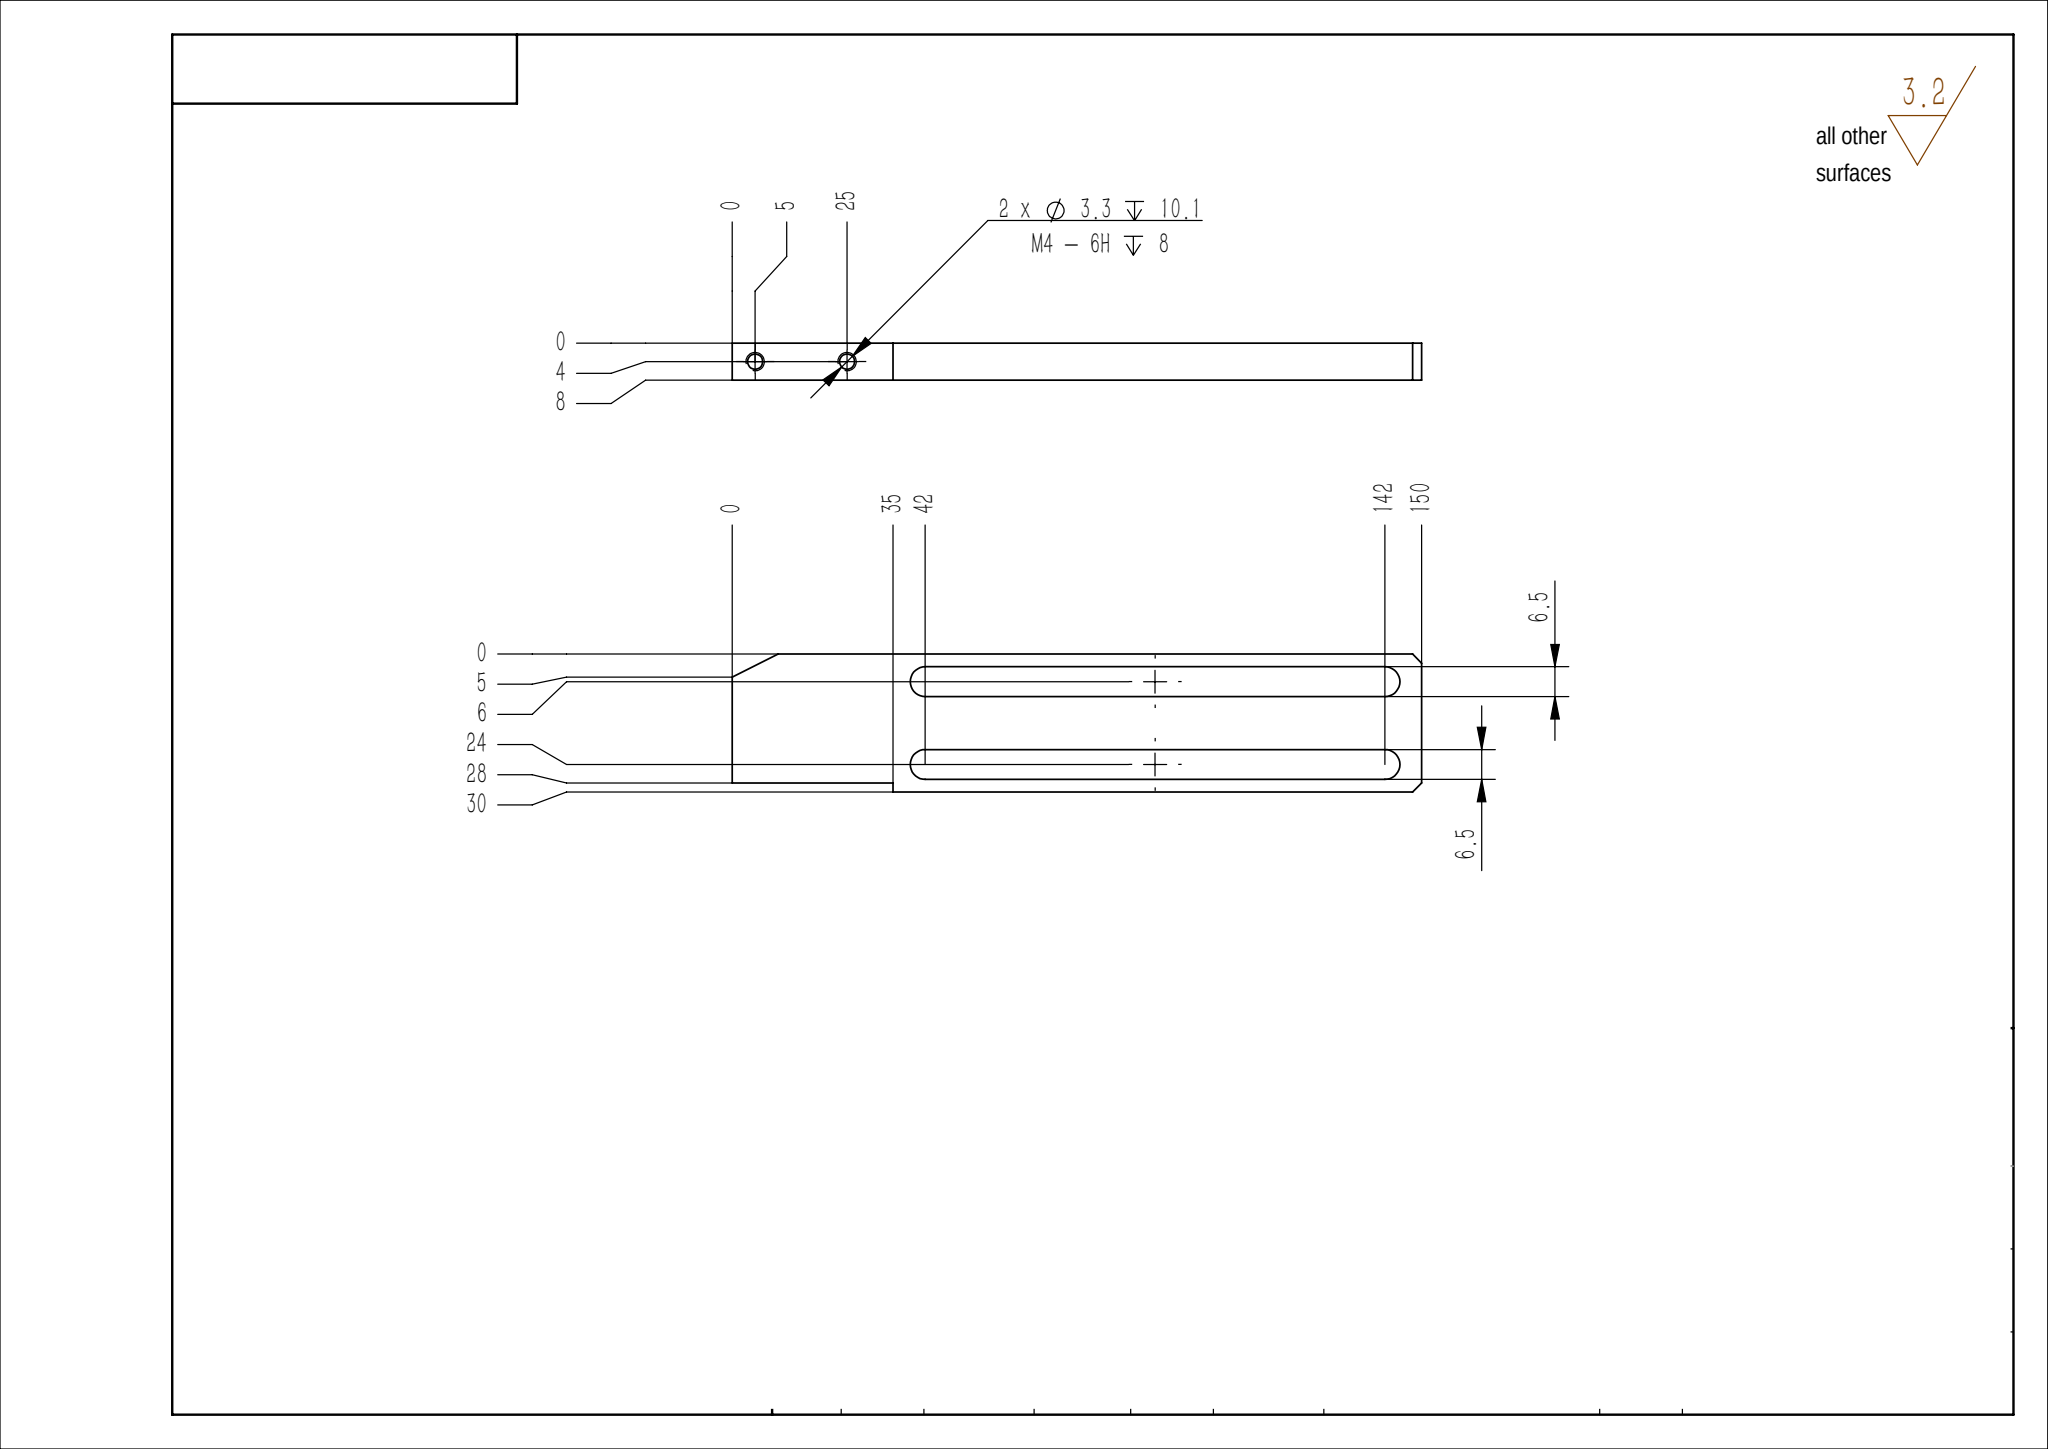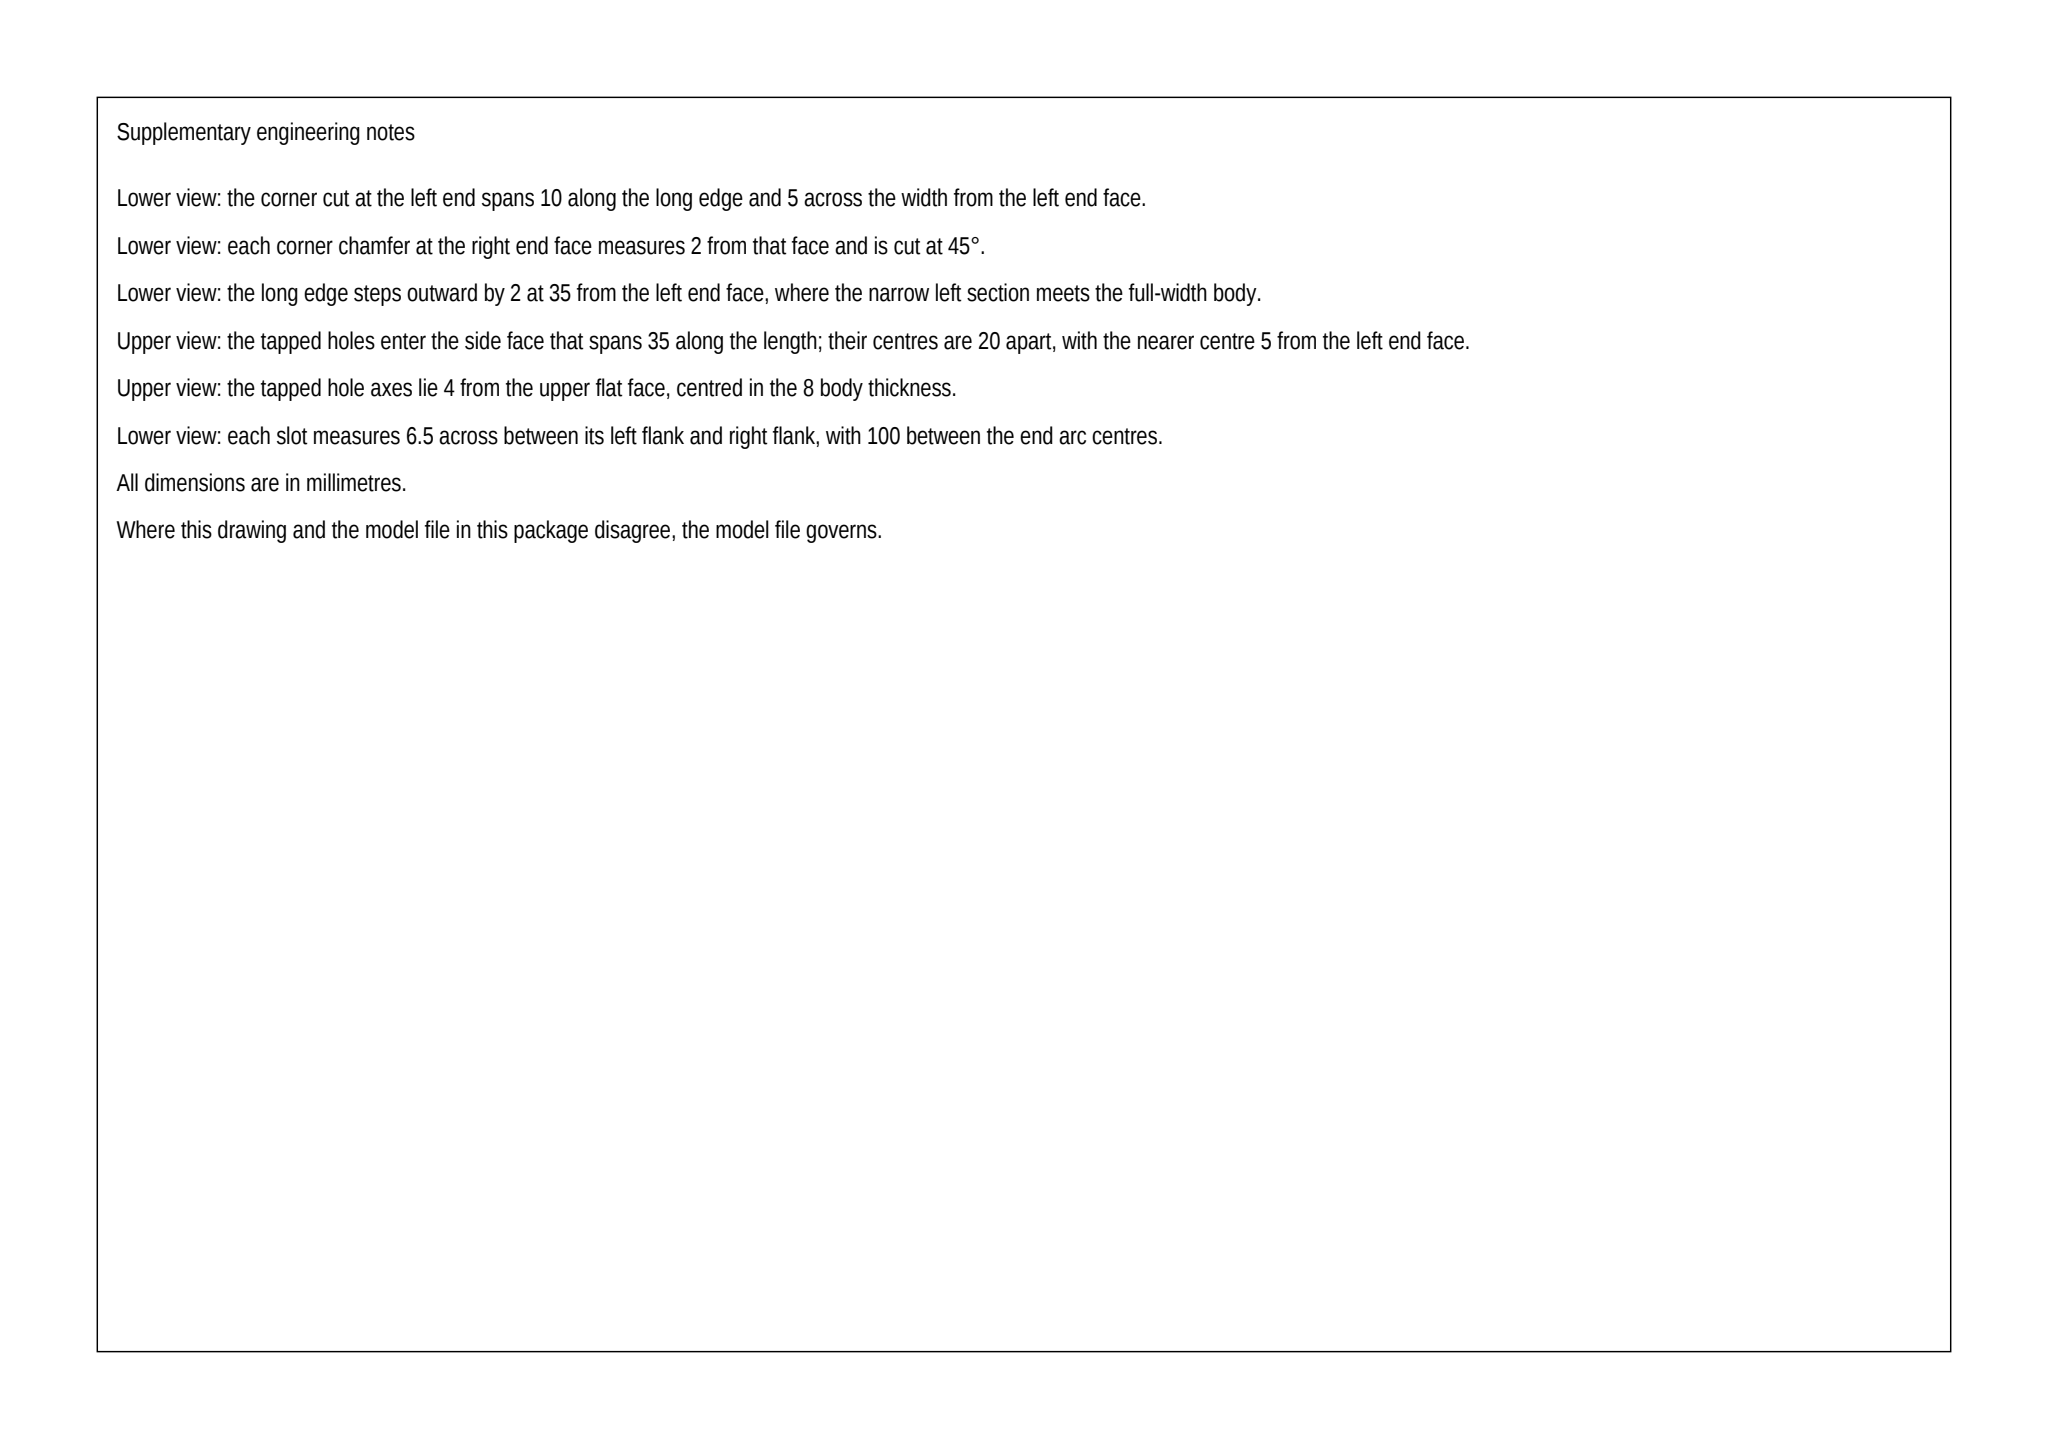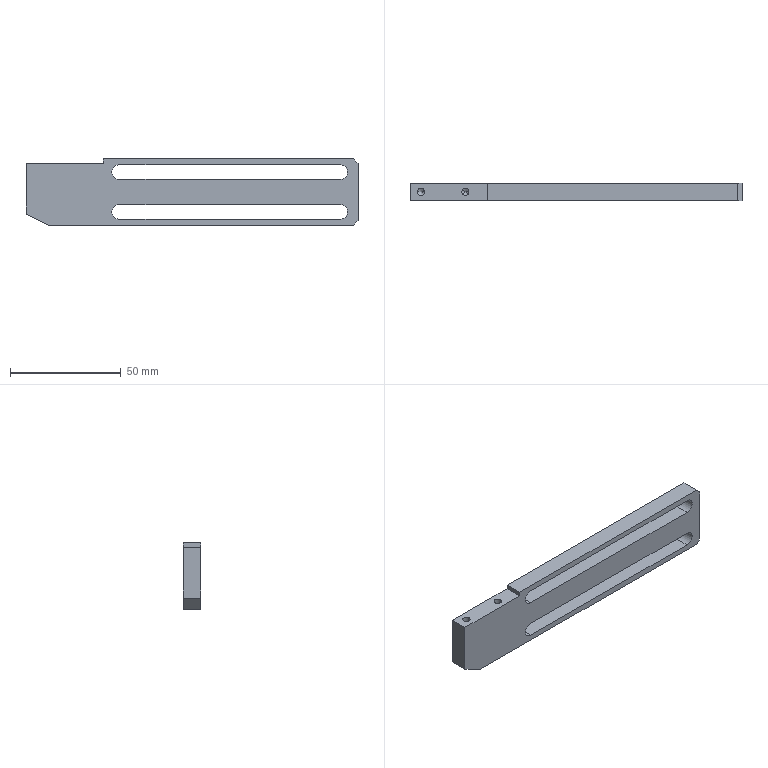Part | SolidWorks | mm | 1 solid | 27 faces | box 150 x 8 x 30 mm | volume 24099 mm3 | plane 15 | cylinder 8 | cone 4 | commonest cylinder face diameters 3.3 x4 6.5 x4
build123d program:
from build123d import *

# Parameters (mm, degrees)
BOSS_EXTRUDE1_DEPTH   = 8
CUT_EXTRUDE1_DEPTH    = 129.173
CUT_EXTRUDE2_DEPTH    = 129.173
CHAMFER1_SIZE         = 2
M4_TAPPED_HOLE1_D     = 3.3
M4_TAPPED_HOLE1_DEPTH = 10.1
M4_TAPPED_HOLE1_TIP   = 0.9914


with BuildPart() as part:
    # Sketch1 → Boss-Extrude1 (new body)
    with BuildSketch(Plane(origin=(0, 0, 0), x_dir=(1, 0, 0), z_dir=(0, 1, 0))):
        Polygon((-23.3, 17.65), (126.7, 17.65), (126.7, -12.35), (11.7, -12.35), (11.7, -10.35), (-23.3, -10.35), align=None)
    extrude(amount=BOSS_EXTRUDE1_DEPTH)

    # Sketch2 → Cut-Extrude1 (cut, through all)
    with BuildSketch(Plane(origin=(0, 8, 0), x_dir=(1, 0, 0), z_dir=(0, 1, 0))):
        with BuildLine():
            Line((18.7, 14.9), (118.7, 14.9))
            ThreePointArc((118.7, 14.9), (121.95, 11.65), (118.7, 8.4))
            Line((118.7, 8.4), (18.7, 8.4))
            ThreePointArc((18.7, 8.4), (15.45, 11.65), (18.7, 14.9))
        make_face()
        with BuildLine():
            Line((18.7, -9.6), (118.7, -9.6))
            ThreePointArc((118.7, -9.6), (121.95, -6.35), (118.7, -3.1))
            Line((118.7, -3.1), (18.7, -3.1))
            ThreePointArc((18.7, -3.1), (15.45, -6.35), (18.7, -9.6))
        make_face()
    extrude(amount=-CUT_EXTRUDE1_DEPTH, mode=Mode.SUBTRACT)

    # Sketch3 → Cut-Extrude2 (cut, through all)
    with BuildSketch(Plane(origin=(0, 8, 0), x_dir=(1, 0, 0), z_dir=(0, 1, 0))):
        Polygon((-23.3, 12.65), (-23.3, 17.65), (-13.3, 17.65), align=None)
    extrude(amount=-CUT_EXTRUDE2_DEPTH, mode=Mode.SUBTRACT)

    # Chamfer1
    chamfer1_edges = [part.edges().sort_by_distance(p)[0] for p in [
        (126.7, 4, -17.65),
        (126.7, 4, 12.35),
    ]]
    chamfer(chamfer1_edges, length=CHAMFER1_SIZE)

    # M4 Tapped Hole1
    with Locations(Plane.XY.offset(10.35)):
        with Locations((-18.3, 4), (1.7, 4)):
            Hole(M4_TAPPED_HOLE1_D / 2, depth=M4_TAPPED_HOLE1_DEPTH)
            with Locations((0, 0, -(M4_TAPPED_HOLE1_DEPTH + M4_TAPPED_HOLE1_TIP / 2))):  # 118° drill point
                Cone(0, M4_TAPPED_HOLE1_D / 2, M4_TAPPED_HOLE1_TIP, mode=Mode.SUBTRACT)


solid = part.part
STEP:
#1=CARTESIAN_POINT('',(-19.95,4.,0.25));
#2=VERTEX_POINT('',#1);
#3=CARTESIAN_POINT('',(-16.65,4.,0.25));
#4=VERTEX_POINT('',#3);
#5=CARTESIAN_POINT('',(-18.3,4.,0.25));
#6=DIRECTION('',(0.,0.,1.));
#7=DIRECTION('',(1.,0.,0.));
#8=AXIS2_PLACEMENT_3D('',#5,#6,#7);
#9=CIRCLE('',#8,1.65);
#10=EDGE_CURVE('',#2,#4,#9,.T.);
#11=ORIENTED_EDGE('',*,*,#10,.F.);
#12=CARTESIAN_POINT('',(-19.95,4.,10.35));
#13=VERTEX_POINT('',#12);
#14=CARTESIAN_POINT('',(-19.95,4.,10.35));
#15=DIRECTION('',(0.,0.,1.));
#16=VECTOR('',#15,1000.);
#17=LINE('',#14,#16);
#18=EDGE_CURVE('',#2,#13,#17,.T.);
#19=ORIENTED_EDGE('',*,*,#18,.T.);
#20=CARTESIAN_POINT('',(-16.65,4.,10.35));
#21=VERTEX_POINT('',#20);
#22=CARTESIAN_POINT('',(-18.3,4.,10.35));
#23=DIRECTION('',(0.,0.,1.));
#24=DIRECTION('',(1.,0.,0.));
#25=AXIS2_PLACEMENT_3D('',#22,#23,#24);
#26=CIRCLE('',#25,1.65);
#27=EDGE_CURVE('',#13,#21,#26,.T.);
#28=ORIENTED_EDGE('',*,*,#27,.T.);
#29=CARTESIAN_POINT('',(-16.65,4.,10.35));
#30=DIRECTION('',(0.,0.,1.));
#31=VECTOR('',#30,1000.);
#32=LINE('',#29,#31);
#33=EDGE_CURVE('',#4,#21,#32,.T.);
#34=ORIENTED_EDGE('',*,*,#33,.F.);
#35=EDGE_LOOP('',(#11,#19,#28,#34));
#36=FACE_OUTER_BOUND('',#35,.T.);
#37=CARTESIAN_POINT('',(-18.3,4.,10.35));
#38=DIRECTION('',(0.,0.,1.));
#39=DIRECTION('',(1.,0.,0.));
#40=AXIS2_PLACEMENT_3D('',#37,#38,#39);
#41=CYLINDRICAL_SURFACE('',#40,1.65);
#42=ADVANCED_FACE('',(#36),#41,.F.);
#43=CARTESIAN_POINT('',(-18.3,4.,-0.7414));
#44=VERTEX_POINT('',#43);
#45=CARTESIAN_POINT('',(-16.65,4.,0.25));
#46=DIRECTION('',(0.8572,0.,0.515));
#47=VECTOR('',#46,1000.);
#48=LINE('',#45,#47);
#49=EDGE_CURVE('',#44,#4,#48,.T.);
#50=ORIENTED_EDGE('',*,*,#49,.F.);
#51=CARTESIAN_POINT('',(-19.95,4.,0.25));
#52=DIRECTION('',(-0.8572,0.,0.515));
#53=VECTOR('',#52,1000.);
#54=LINE('',#51,#53);
#55=EDGE_CURVE('',#44,#2,#54,.T.);
#56=ORIENTED_EDGE('',*,*,#55,.T.);
#57=ORIENTED_EDGE('',*,*,#10,.T.);
#58=EDGE_LOOP('',(#50,#56,#57));
#59=FACE_OUTER_BOUND('',#58,.T.);
#60=CARTESIAN_POINT('',(-18.3,4.,0.25));
#61=DIRECTION('',(0.,0.,1.));
#62=DIRECTION('',(1.,0.,0.));
#63=AXIS2_PLACEMENT_3D('',#60,#61,#62);
#64=CONICAL_SURFACE('',#63,1.65,1.03);
#65=ADVANCED_FACE('',(#59),#64,.F.);
#66=CARTESIAN_POINT('',(0.05,4.,0.25));
#67=VERTEX_POINT('',#66);
#68=CARTESIAN_POINT('',(3.35,4.,0.25));
#69=VERTEX_POINT('',#68);
#70=CARTESIAN_POINT('',(1.7,4.,0.25));
#71=DIRECTION('',(0.,0.,1.));
#72=DIRECTION('',(1.,0.,0.));
#73=AXIS2_PLACEMENT_3D('',#70,#71,#72);
#74=CIRCLE('',#73,1.65);
#75=EDGE_CURVE('',#67,#69,#74,.T.);
#76=ORIENTED_EDGE('',*,*,#75,.F.);
#77=CARTESIAN_POINT('',(0.05,4.,10.35));
#78=VERTEX_POINT('',#77);
#79=CARTESIAN_POINT('',(0.05,4.,10.35));
#80=DIRECTION('',(0.,0.,1.));
#81=VECTOR('',#80,1000.);
#82=LINE('',#79,#81);
#83=EDGE_CURVE('',#67,#78,#82,.T.);
#84=ORIENTED_EDGE('',*,*,#83,.T.);
#85=CARTESIAN_POINT('',(3.35,4.,10.35));
#86=VERTEX_POINT('',#85);
#87=CARTESIAN_POINT('',(1.7,4.,10.35));
#88=DIRECTION('',(0.,0.,1.));
#89=DIRECTION('',(1.,0.,0.));
#90=AXIS2_PLACEMENT_3D('',#87,#88,#89);
#91=CIRCLE('',#90,1.65);
#92=EDGE_CURVE('',#78,#86,#91,.T.);
#93=ORIENTED_EDGE('',*,*,#92,.T.);
#94=CARTESIAN_POINT('',(3.35,4.,10.35));
#95=DIRECTION('',(0.,0.,1.));
#96=VECTOR('',#95,1000.);
#97=LINE('',#94,#96);
#98=EDGE_CURVE('',#69,#86,#97,.T.);
#99=ORIENTED_EDGE('',*,*,#98,.F.);
#100=EDGE_LOOP('',(#76,#84,#93,#99));
#101=FACE_OUTER_BOUND('',#100,.T.);
#102=CARTESIAN_POINT('',(1.7,4.,10.35));
#103=DIRECTION('',(0.,0.,1.));
#104=DIRECTION('',(1.,0.,0.));
#105=AXIS2_PLACEMENT_3D('',#102,#103,#104);
#106=CYLINDRICAL_SURFACE('',#105,1.65);
#107=ADVANCED_FACE('',(#101),#106,.F.);
#108=CARTESIAN_POINT('',(1.7,4.,-0.7414));
#109=VERTEX_POINT('',#108);
#110=CARTESIAN_POINT('',(3.35,4.,0.25));
#111=DIRECTION('',(0.8572,0.,0.515));
#112=VECTOR('',#111,1000.);
#113=LINE('',#110,#112);
#114=EDGE_CURVE('',#109,#69,#113,.T.);
#115=ORIENTED_EDGE('',*,*,#114,.F.);
#116=CARTESIAN_POINT('',(0.05,4.,0.25));
#117=DIRECTION('',(-0.8572,0.,0.515));
#118=VECTOR('',#117,1000.);
#119=LINE('',#116,#118);
#120=EDGE_CURVE('',#109,#67,#119,.T.);
#121=ORIENTED_EDGE('',*,*,#120,.T.);
#122=ORIENTED_EDGE('',*,*,#75,.T.);
#123=EDGE_LOOP('',(#115,#121,#122));
#124=FACE_OUTER_BOUND('',#123,.T.);
#125=CARTESIAN_POINT('',(1.7,4.,0.25));
#126=DIRECTION('',(0.,0.,1.));
#127=DIRECTION('',(1.,0.,0.));
#128=AXIS2_PLACEMENT_3D('',#125,#126,#127);
#129=CONICAL_SURFACE('',#128,1.65,1.03);
#130=ADVANCED_FACE('',(#124),#129,.F.);
#131=CARTESIAN_POINT('',(-23.3,8.,-12.65));
#132=VERTEX_POINT('',#131);
#133=CARTESIAN_POINT('',(-23.3,8.,10.35));
#134=VERTEX_POINT('',#133);
#135=CARTESIAN_POINT('',(-23.3,8.,10.35));
#136=DIRECTION('',(0.,0.,1.));
#137=VECTOR('',#136,1000.);
#138=LINE('',#135,#137);
#139=EDGE_CURVE('',#132,#134,#138,.T.);
#140=ORIENTED_EDGE('',*,*,#139,.F.);
#141=CARTESIAN_POINT('',(-23.3,0.,-12.65));
#142=VERTEX_POINT('',#141);
#143=CARTESIAN_POINT('',(-23.3,0.,-12.65));
#144=DIRECTION('',(0.,1.,0.));
#145=VECTOR('',#144,1000.);
#146=LINE('',#143,#145);
#147=EDGE_CURVE('',#142,#132,#146,.T.);
#148=ORIENTED_EDGE('',*,*,#147,.F.);
#149=CARTESIAN_POINT('',(-23.3,0.,10.35));
#150=VERTEX_POINT('',#149);
#151=CARTESIAN_POINT('',(-23.3,0.,10.35));
#152=DIRECTION('',(0.,0.,1.));
#153=VECTOR('',#152,1000.);
#154=LINE('',#151,#153);
#155=EDGE_CURVE('',#142,#150,#154,.T.);
#156=ORIENTED_EDGE('',*,*,#155,.T.);
#157=CARTESIAN_POINT('',(-23.3,8.,10.35));
#158=DIRECTION('',(0.,-1.,0.));
#159=VECTOR('',#158,1000.);
#160=LINE('',#157,#159);
#161=EDGE_CURVE('',#134,#150,#160,.T.);
#162=ORIENTED_EDGE('',*,*,#161,.F.);
#163=EDGE_LOOP('',(#140,#148,#156,#162));
#164=FACE_OUTER_BOUND('',#163,.T.);
#165=CARTESIAN_POINT('',(-23.3,8.,10.35));
#166=DIRECTION('',(1.,0.,-0.));
#167=DIRECTION('',(-0.,0.,-1.));
#168=AXIS2_PLACEMENT_3D('',#165,#166,#167);
#169=PLANE('',#168);
#170=ADVANCED_FACE('',(#164),#169,.F.);
#171=CARTESIAN_POINT('',(-18.3,4.,10.35));
#172=DIRECTION('',(0.,0.,1.));
#173=DIRECTION('',(1.,0.,0.));
#174=AXIS2_PLACEMENT_3D('',#171,#172,#173);
#175=CIRCLE('',#174,1.65);
#176=EDGE_CURVE('',#21,#13,#175,.T.);
#177=ORIENTED_EDGE('',*,*,#176,.F.);
#178=ORIENTED_EDGE('',*,*,#27,.F.);
#179=EDGE_LOOP('',(#177,#178));
#180=FACE_BOUND('',#179,.T.);
#181=CARTESIAN_POINT('',(1.7,4.,10.35));
#182=DIRECTION('',(0.,0.,1.));
#183=DIRECTION('',(1.,0.,0.));
#184=AXIS2_PLACEMENT_3D('',#181,#182,#183);
#185=CIRCLE('',#184,1.65);
#186=EDGE_CURVE('',#86,#78,#185,.T.);
#187=ORIENTED_EDGE('',*,*,#186,.F.);
#188=ORIENTED_EDGE('',*,*,#92,.F.);
#189=EDGE_LOOP('',(#187,#188));
#190=FACE_BOUND('',#189,.T.);
#191=CARTESIAN_POINT('',(11.7,0.,10.35));
#192=VERTEX_POINT('',#191);
#193=CARTESIAN_POINT('',(11.7,0.,10.35));
#194=DIRECTION('',(1.,0.,-0.));
#195=VECTOR('',#194,1000.);
#196=LINE('',#193,#195);
#197=EDGE_CURVE('',#150,#192,#196,.T.);
#198=ORIENTED_EDGE('',*,*,#197,.T.);
#199=CARTESIAN_POINT('',(11.7,8.,10.35));
#200=VERTEX_POINT('',#199);
#201=CARTESIAN_POINT('',(11.7,8.,10.35));
#202=DIRECTION('',(0.,-1.,0.));
#203=VECTOR('',#202,1000.);
#204=LINE('',#201,#203);
#205=EDGE_CURVE('',#200,#192,#204,.T.);
#206=ORIENTED_EDGE('',*,*,#205,.F.);
#207=CARTESIAN_POINT('',(11.7,8.,10.35));
#208=DIRECTION('',(1.,0.,-0.));
#209=VECTOR('',#208,1000.);
#210=LINE('',#207,#209);
#211=EDGE_CURVE('',#134,#200,#210,.T.);
#212=ORIENTED_EDGE('',*,*,#211,.F.);
#213=ORIENTED_EDGE('',*,*,#161,.T.);
#214=EDGE_LOOP('',(#198,#206,#212,#213));
#215=FACE_OUTER_BOUND('',#214,.T.);
#216=CARTESIAN_POINT('',(11.7,8.,10.35));
#217=DIRECTION('',(-0.,0.,-1.));
#218=DIRECTION('',(-1.,0.,0.));
#219=AXIS2_PLACEMENT_3D('',#216,#217,#218);
#220=PLANE('',#219);
#221=ADVANCED_FACE('',(#180,#190,#215),#220,.F.);
#222=CARTESIAN_POINT('',(11.7,0.,12.35));
#223=VERTEX_POINT('',#222);
#224=CARTESIAN_POINT('',(11.7,0.,12.35));
#225=DIRECTION('',(0.,0.,1.));
#226=VECTOR('',#225,1000.);
#227=LINE('',#224,#226);
#228=EDGE_CURVE('',#192,#223,#227,.T.);
#229=ORIENTED_EDGE('',*,*,#228,.T.);
#230=CARTESIAN_POINT('',(11.7,8.,12.35));
#231=VERTEX_POINT('',#230);
#232=CARTESIAN_POINT('',(11.7,8.,12.35));
#233=DIRECTION('',(0.,-1.,0.));
#234=VECTOR('',#233,1000.);
#235=LINE('',#232,#234);
#236=EDGE_CURVE('',#231,#223,#235,.T.);
#237=ORIENTED_EDGE('',*,*,#236,.F.);
#238=CARTESIAN_POINT('',(11.7,8.,12.35));
#239=DIRECTION('',(0.,0.,1.));
#240=VECTOR('',#239,1000.);
#241=LINE('',#238,#240);
#242=EDGE_CURVE('',#200,#231,#241,.T.);
#243=ORIENTED_EDGE('',*,*,#242,.F.);
#244=ORIENTED_EDGE('',*,*,#205,.T.);
#245=EDGE_LOOP('',(#229,#237,#243,#244));
#246=FACE_OUTER_BOUND('',#245,.T.);
#247=CARTESIAN_POINT('',(11.7,8.,12.35));
#248=DIRECTION('',(1.,0.,0.));
#249=DIRECTION('',(0.,0.,-1.));
#250=AXIS2_PLACEMENT_3D('',#247,#248,#249);
#251=PLANE('',#250);
#252=ADVANCED_FACE('',(#246),#251,.F.);
#253=CARTESIAN_POINT('',(124.7,0.,12.35));
#254=VERTEX_POINT('',#253);
#255=CARTESIAN_POINT('',(126.7,0.,12.35));
#256=DIRECTION('',(1.,0.,-0.));
#257=VECTOR('',#256,1000.);
#258=LINE('',#255,#257);
#259=EDGE_CURVE('',#223,#254,#258,.T.);
#260=ORIENTED_EDGE('',*,*,#259,.T.);
#261=CARTESIAN_POINT('',(124.7,8.,12.35));
#262=VERTEX_POINT('',#261);
#263=CARTESIAN_POINT('',(124.7,8.,12.35));
#264=DIRECTION('',(0.,1.,0.));
#265=VECTOR('',#264,1000.);
#266=LINE('',#263,#265);
#267=EDGE_CURVE('',#254,#262,#266,.T.);
#268=ORIENTED_EDGE('',*,*,#267,.T.);
#269=CARTESIAN_POINT('',(126.7,8.,12.35));
#270=DIRECTION('',(1.,0.,-0.));
#271=VECTOR('',#270,1000.);
#272=LINE('',#269,#271);
#273=EDGE_CURVE('',#231,#262,#272,.T.);
#274=ORIENTED_EDGE('',*,*,#273,.F.);
#275=ORIENTED_EDGE('',*,*,#236,.T.);
#276=EDGE_LOOP('',(#260,#268,#274,#275));
#277=FACE_OUTER_BOUND('',#276,.T.);
#278=CARTESIAN_POINT('',(126.7,8.,12.35));
#279=DIRECTION('',(-0.,0.,-1.));
#280=DIRECTION('',(-1.,0.,0.));
#281=AXIS2_PLACEMENT_3D('',#278,#279,#280);
#282=PLANE('',#281);
#283=ADVANCED_FACE('',(#277),#282,.F.);
#284=CARTESIAN_POINT('',(126.7,8.,10.35));
#285=VERTEX_POINT('',#284);
#286=CARTESIAN_POINT('',(126.7,8.,-15.65));
#287=VERTEX_POINT('',#286);
#288=CARTESIAN_POINT('',(126.7,8.,-17.65));
#289=DIRECTION('',(0.,0.,-1.));
#290=VECTOR('',#289,1000.);
#291=LINE('',#288,#290);
#292=EDGE_CURVE('',#285,#287,#291,.T.);
#293=ORIENTED_EDGE('',*,*,#292,.F.);
#294=CARTESIAN_POINT('',(126.7,0.,10.35));
#295=VERTEX_POINT('',#294);
#296=CARTESIAN_POINT('',(126.7,8.,10.35));
#297=DIRECTION('',(0.,-1.,0.));
#298=VECTOR('',#297,1000.);
#299=LINE('',#296,#298);
#300=EDGE_CURVE('',#285,#295,#299,.T.);
#301=ORIENTED_EDGE('',*,*,#300,.T.);
#302=CARTESIAN_POINT('',(126.7,0.,-15.65));
#303=VERTEX_POINT('',#302);
#304=CARTESIAN_POINT('',(126.7,0.,-17.65));
#305=DIRECTION('',(0.,0.,-1.));
#306=VECTOR('',#305,1000.);
#307=LINE('',#304,#306);
#308=EDGE_CURVE('',#295,#303,#307,.T.);
#309=ORIENTED_EDGE('',*,*,#308,.T.);
#310=CARTESIAN_POINT('',(126.7,8.,-15.65));
#311=DIRECTION('',(0.,1.,0.));
#312=VECTOR('',#311,1000.);
#313=LINE('',#310,#312);
#314=EDGE_CURVE('',#303,#287,#313,.T.);
#315=ORIENTED_EDGE('',*,*,#314,.T.);
#316=EDGE_LOOP('',(#293,#301,#309,#315));
#317=FACE_OUTER_BOUND('',#316,.T.);
#318=CARTESIAN_POINT('',(126.7,8.,-17.65));
#319=DIRECTION('',(-1.,0.,0.));
#320=DIRECTION('',(0.,0.,1.));
#321=AXIS2_PLACEMENT_3D('',#318,#319,#320);
#322=PLANE('',#321);
#323=ADVANCED_FACE('',(#317),#322,.F.);
#324=CARTESIAN_POINT('',(124.7,8.,-17.65));
#325=VERTEX_POINT('',#324);
#326=CARTESIAN_POINT('',(-13.3,8.,-17.65));
#327=VERTEX_POINT('',#326);
#328=CARTESIAN_POINT('',(-23.3,8.,-17.65));
#329=DIRECTION('',(-1.,0.,0.));
#330=VECTOR('',#329,1000.);
#331=LINE('',#328,#330);
#332=EDGE_CURVE('',#325,#327,#331,.T.);
#333=ORIENTED_EDGE('',*,*,#332,.F.);
#334=CARTESIAN_POINT('',(124.7,0.,-17.65));
#335=VERTEX_POINT('',#334);
#336=CARTESIAN_POINT('',(124.7,8.,-17.65));
#337=DIRECTION('',(0.,-1.,0.));
#338=VECTOR('',#337,1000.);
#339=LINE('',#336,#338);
#340=EDGE_CURVE('',#325,#335,#339,.T.);
#341=ORIENTED_EDGE('',*,*,#340,.T.);
#342=CARTESIAN_POINT('',(-13.3,0.,-17.65));
#343=VERTEX_POINT('',#342);
#344=CARTESIAN_POINT('',(-23.3,0.,-17.65));
#345=DIRECTION('',(-1.,0.,0.));
#346=VECTOR('',#345,1000.);
#347=LINE('',#344,#346);
#348=EDGE_CURVE('',#335,#343,#347,.T.);
#349=ORIENTED_EDGE('',*,*,#348,.T.);
#350=CARTESIAN_POINT('',(-13.3,0.,-17.65));
#351=DIRECTION('',(0.,1.,0.));
#352=VECTOR('',#351,1000.);
#353=LINE('',#350,#352);
#354=EDGE_CURVE('',#343,#327,#353,.T.);
#355=ORIENTED_EDGE('',*,*,#354,.T.);
#356=EDGE_LOOP('',(#333,#341,#349,#355));
#357=FACE_OUTER_BOUND('',#356,.T.);
#358=CARTESIAN_POINT('',(-23.3,8.,-17.65));
#359=DIRECTION('',(0.,0.,1.));
#360=DIRECTION('',(1.,0.,-0.));
#361=AXIS2_PLACEMENT_3D('',#358,#359,#360);
#362=PLANE('',#361);
#363=ADVANCED_FACE('',(#357),#362,.F.);
#364=CARTESIAN_POINT('',(18.7,8.,9.6));
#365=VERTEX_POINT('',#364);
#366=CARTESIAN_POINT('',(118.7,8.,9.6));
#367=VERTEX_POINT('',#366);
#368=CARTESIAN_POINT('',(18.7,8.,9.6));
#369=DIRECTION('',(1.,0.,0.));
#370=VECTOR('',#369,1000.);
#371=LINE('',#368,#370);
#372=EDGE_CURVE('',#365,#367,#371,.T.);
#373=ORIENTED_EDGE('',*,*,#372,.F.);
#374=CARTESIAN_POINT('',(18.7,8.,3.1));
#375=VERTEX_POINT('',#374);
#376=CARTESIAN_POINT('',(18.7,8.,6.35));
#377=DIRECTION('',(0.,1.,0.));
#378=DIRECTION('',(0.,0.,-1.));
#379=AXIS2_PLACEMENT_3D('',#376,#377,#378);
#380=CIRCLE('',#379,3.25);
#381=EDGE_CURVE('',#375,#365,#380,.T.);
#382=ORIENTED_EDGE('',*,*,#381,.F.);
#383=CARTESIAN_POINT('',(118.7,8.,3.1));
#384=VERTEX_POINT('',#383);
#385=CARTESIAN_POINT('',(18.7,8.,3.1));
#386=DIRECTION('',(-1.,0.,0.));
#387=VECTOR('',#386,1000.);
#388=LINE('',#385,#387);
#389=EDGE_CURVE('',#384,#375,#388,.T.);
#390=ORIENTED_EDGE('',*,*,#389,.F.);
#391=CARTESIAN_POINT('',(118.7,8.,6.35));
#392=DIRECTION('',(0.,1.,0.));
#393=DIRECTION('',(0.,0.,-1.));
#394=AXIS2_PLACEMENT_3D('',#391,#392,#393);
#395=CIRCLE('',#394,3.25);
#396=EDGE_CURVE('',#367,#384,#395,.T.);
#397=ORIENTED_EDGE('',*,*,#396,.F.);
#398=EDGE_LOOP('',(#373,#382,#390,#397));
#399=FACE_BOUND('',#398,.T.);
#400=CARTESIAN_POINT('',(18.7,8.,-8.4));
#401=VERTEX_POINT('',#400);
#402=CARTESIAN_POINT('',(118.7,8.,-8.4));
#403=VERTEX_POINT('',#402);
#404=CARTESIAN_POINT('',(18.7,8.,-8.4));
#405=DIRECTION('',(1.,0.,0.));
#406=VECTOR('',#405,1000.);
#407=LINE('',#404,#406);
#408=EDGE_CURVE('',#401,#403,#407,.T.);
#409=ORIENTED_EDGE('',*,*,#408,.F.);
#410=CARTESIAN_POINT('',(18.7,8.,-14.9));
#411=VERTEX_POINT('',#410);
#412=CARTESIAN_POINT('',(18.7,8.,-11.65));
#413=DIRECTION('',(0.,1.,0.));
#414=DIRECTION('',(0.,0.,1.));
#415=AXIS2_PLACEMENT_3D('',#412,#413,#414);
#416=CIRCLE('',#415,3.25);
#417=EDGE_CURVE('',#411,#401,#416,.T.);
#418=ORIENTED_EDGE('',*,*,#417,.F.);
#419=CARTESIAN_POINT('',(118.7,8.,-14.9));
#420=VERTEX_POINT('',#419);
#421=CARTESIAN_POINT('',(18.7,8.,-14.9));
#422=DIRECTION('',(-1.,0.,0.));
#423=VECTOR('',#422,1000.);
#424=LINE('',#421,#423);
#425=EDGE_CURVE('',#420,#411,#424,.T.);
#426=ORIENTED_EDGE('',*,*,#425,.F.);
#427=CARTESIAN_POINT('',(118.7,8.,-11.65));
#428=DIRECTION('',(0.,1.,0.));
#429=DIRECTION('',(0.,0.,1.));
#430=AXIS2_PLACEMENT_3D('',#427,#428,#429);
#431=CIRCLE('',#430,3.25);
#432=EDGE_CURVE('',#403,#420,#431,.T.);
#433=ORIENTED_EDGE('',*,*,#432,.F.);
#434=EDGE_LOOP('',(#409,#418,#426,#433));
#435=FACE_BOUND('',#434,.T.);
#436=ORIENTED_EDGE('',*,*,#273,.T.);
#437=CARTESIAN_POINT('',(126.7,8.,10.35));
#438=DIRECTION('',(0.7071,0.,-0.7071));
#439=VECTOR('',#438,1000.);
#440=LINE('',#437,#439);
#441=EDGE_CURVE('',#262,#285,#440,.T.);
#442=ORIENTED_EDGE('',*,*,#441,.T.);
#443=ORIENTED_EDGE('',*,*,#292,.T.);
#444=CARTESIAN_POINT('',(124.7,8.,-17.65));
#445=DIRECTION('',(-0.7071,0.,-0.7071));
#446=VECTOR('',#445,1000.);
#447=LINE('',#444,#446);
#448=EDGE_CURVE('',#287,#325,#447,.T.);
#449=ORIENTED_EDGE('',*,*,#448,.T.);
#450=ORIENTED_EDGE('',*,*,#332,.T.);
#451=CARTESIAN_POINT('',(-13.3,8.,-17.65));
#452=DIRECTION('',(0.8944,0.,-0.4472));
#453=VECTOR('',#452,1000.);
#454=LINE('',#451,#453);
#455=EDGE_CURVE('',#132,#327,#454,.T.);
#456=ORIENTED_EDGE('',*,*,#455,.F.);
#457=ORIENTED_EDGE('',*,*,#139,.T.);
#458=ORIENTED_EDGE('',*,*,#211,.T.);
#459=ORIENTED_EDGE('',*,*,#242,.T.);
#460=EDGE_LOOP('',(#436,#442,#443,#449,#450,#456,#457,#458,#459));
#461=FACE_OUTER_BOUND('',#460,.T.);
#462=CARTESIAN_POINT('',(0.,8.,0.));
#463=DIRECTION('',(0.,-1.,0.));
#464=DIRECTION('',(0.,0.,-1.));
#465=AXIS2_PLACEMENT_3D('',#462,#463,#464);
#466=PLANE('',#465);
#467=ADVANCED_FACE('',(#399,#435,#461),#466,.F.);
#468=ORIENTED_EDGE('',*,*,#308,.F.);
#469=CARTESIAN_POINT('',(68.525,0.,68.525));
#470=DIRECTION('',(-0.7071,0.,0.7071));
#471=VECTOR('',#470,1000.);
#472=LINE('',#469,#471);
#473=EDGE_CURVE('',#295,#254,#472,.T.);
#474=ORIENTED_EDGE('',*,*,#473,.T.);
#475=ORIENTED_EDGE('',*,*,#259,.F.);
#476=ORIENTED_EDGE('',*,*,#228,.F.);
#477=ORIENTED_EDGE('',*,*,#197,.F.);
#478=ORIENTED_EDGE('',*,*,#155,.F.);
#479=CARTESIAN_POINT('',(-13.3,0.,-17.65));
#480=DIRECTION('',(0.8944,0.,-0.4472));
#481=VECTOR('',#480,1000.);
#482=LINE('',#479,#481);
#483=EDGE_CURVE('',#142,#343,#482,.T.);
#484=ORIENTED_EDGE('',*,*,#483,.T.);
#485=ORIENTED_EDGE('',*,*,#348,.F.);
#486=CARTESIAN_POINT('',(71.175,0.,-71.175));
#487=DIRECTION('',(0.7071,0.,0.7071));
#488=VECTOR('',#487,1000.);
#489=LINE('',#486,#488);
#490=EDGE_CURVE('',#335,#303,#489,.T.);
#491=ORIENTED_EDGE('',*,*,#490,.T.);
#492=EDGE_LOOP('',(#468,#474,#475,#476,#477,#478,#484,#485,#491));
#493=FACE_OUTER_BOUND('',#492,.T.);
#494=CARTESIAN_POINT('',(18.7,0.,3.1));
#495=VERTEX_POINT('',#494);
#496=CARTESIAN_POINT('',(18.7,0.,9.6));
#497=VERTEX_POINT('',#496);
#498=CARTESIAN_POINT('',(18.7,0.,6.35));
#499=DIRECTION('',(0.,1.,0.));
#500=DIRECTION('',(0.,0.,-1.));
#501=AXIS2_PLACEMENT_3D('',#498,#499,#500);
#502=CIRCLE('',#501,3.25);
#503=EDGE_CURVE('',#495,#497,#502,.T.);
#504=ORIENTED_EDGE('',*,*,#503,.T.);
#505=CARTESIAN_POINT('',(118.7,0.,9.6));
#506=VERTEX_POINT('',#505);
#507=CARTESIAN_POINT('',(18.7,0.,9.6));
#508=DIRECTION('',(1.,0.,0.));
#509=VECTOR('',#508,1000.);
#510=LINE('',#507,#509);
#511=EDGE_CURVE('',#497,#506,#510,.T.);
#512=ORIENTED_EDGE('',*,*,#511,.T.);
#513=CARTESIAN_POINT('',(118.7,0.,3.1));
#514=VERTEX_POINT('',#513);
#515=CARTESIAN_POINT('',(118.7,0.,6.35));
#516=DIRECTION('',(0.,1.,0.));
#517=DIRECTION('',(0.,0.,-1.));
#518=AXIS2_PLACEMENT_3D('',#515,#516,#517);
#519=CIRCLE('',#518,3.25);
#520=EDGE_CURVE('',#506,#514,#519,.T.);
#521=ORIENTED_EDGE('',*,*,#520,.T.);
#522=CARTESIAN_POINT('',(18.7,0.,3.1));
#523=DIRECTION('',(-1.,0.,0.));
#524=VECTOR('',#523,1000.);
#525=LINE('',#522,#524);
#526=EDGE_CURVE('',#514,#495,#525,.T.);
#527=ORIENTED_EDGE('',*,*,#526,.T.);
#528=EDGE_LOOP('',(#504,#512,#521,#527));
#529=FACE_BOUND('',#528,.T.);
#530=CARTESIAN_POINT('',(18.7,0.,-14.9));
#531=VERTEX_POINT('',#530);
#532=CARTESIAN_POINT('',(18.7,0.,-8.4));
#533=VERTEX_POINT('',#532);
#534=CARTESIAN_POINT('',(18.7,0.,-11.65));
#535=DIRECTION('',(0.,1.,0.));
#536=DIRECTION('',(0.,0.,1.));
#537=AXIS2_PLACEMENT_3D('',#534,#535,#536);
#538=CIRCLE('',#537,3.25);
#539=EDGE_CURVE('',#531,#533,#538,.T.);
#540=ORIENTED_EDGE('',*,*,#539,.T.);
#541=CARTESIAN_POINT('',(118.7,0.,-8.4));
#542=VERTEX_POINT('',#541);
#543=CARTESIAN_POINT('',(18.7,0.,-8.4));
#544=DIRECTION('',(1.,0.,0.));
#545=VECTOR('',#544,1000.);
#546=LINE('',#543,#545);
#547=EDGE_CURVE('',#533,#542,#546,.T.);
#548=ORIENTED_EDGE('',*,*,#547,.T.);
#549=CARTESIAN_POINT('',(118.7,0.,-14.9));
#550=VERTEX_POINT('',#549);
#551=CARTESIAN_POINT('',(118.7,0.,-11.65));
#552=DIRECTION('',(0.,1.,0.));
#553=DIRECTION('',(0.,0.,1.));
#554=AXIS2_PLACEMENT_3D('',#551,#552,#553);
#555=CIRCLE('',#554,3.25);
#556=EDGE_CURVE('',#542,#550,#555,.T.);
#557=ORIENTED_EDGE('',*,*,#556,.T.);
#558=CARTESIAN_POINT('',(18.7,0.,-14.9));
#559=DIRECTION('',(-1.,0.,0.));
#560=VECTOR('',#559,1000.);
#561=LINE('',#558,#560);
#562=EDGE_CURVE('',#550,#531,#561,.T.);
#563=ORIENTED_EDGE('',*,*,#562,.T.);
#564=EDGE_LOOP('',(#540,#548,#557,#563));
#565=FACE_BOUND('',#564,.T.);
#566=CARTESIAN_POINT('',(0.,0.,0.));
#567=DIRECTION('',(0.,-1.,0.));
#568=DIRECTION('',(0.,0.,-1.));
#569=AXIS2_PLACEMENT_3D('',#566,#567,#568);
#570=PLANE('',#569);
#571=ADVANCED_FACE('',(#493,#529,#565),#570,.T.);
#572=ORIENTED_EDGE('',*,*,#417,.T.);
#573=CARTESIAN_POINT('',(18.7,0.,-8.4));
#574=DIRECTION('',(0.,1.,0.));
#575=VECTOR('',#574,1000.);
#576=LINE('',#573,#575);
#577=EDGE_CURVE('',#533,#401,#576,.T.);
#578=ORIENTED_EDGE('',*,*,#577,.F.);
#579=ORIENTED_EDGE('',*,*,#539,.F.);
#580=CARTESIAN_POINT('',(18.7,0.,-14.9));
#581=DIRECTION('',(0.,1.,0.));
#582=VECTOR('',#581,1000.);
#583=LINE('',#580,#582);
#584=EDGE_CURVE('',#531,#411,#583,.T.);
#585=ORIENTED_EDGE('',*,*,#584,.T.);
#586=EDGE_LOOP('',(#572,#578,#579,#585));
#587=FACE_OUTER_BOUND('',#586,.T.);
#588=CARTESIAN_POINT('',(18.7,0.,-11.65));
#589=DIRECTION('',(0.,1.,0.));
#590=DIRECTION('',(0.,0.,1.));
#591=AXIS2_PLACEMENT_3D('',#588,#589,#590);
#592=CYLINDRICAL_SURFACE('',#591,3.25);
#593=ADVANCED_FACE('',(#587),#592,.F.);
#594=ORIENTED_EDGE('',*,*,#425,.T.);
#595=ORIENTED_EDGE('',*,*,#584,.F.);
#596=ORIENTED_EDGE('',*,*,#562,.F.);
#597=CARTESIAN_POINT('',(118.7,0.,-14.9));
#598=DIRECTION('',(0.,1.,0.));
#599=VECTOR('',#598,1000.);
#600=LINE('',#597,#599);
#601=EDGE_CURVE('',#550,#420,#600,.T.);
#602=ORIENTED_EDGE('',*,*,#601,.T.);
#603=EDGE_LOOP('',(#594,#595,#596,#602));
#604=FACE_OUTER_BOUND('',#603,.T.);
#605=CARTESIAN_POINT('',(18.7,0.,-14.9));
#606=DIRECTION('',(0.,0.,-1.));
#607=DIRECTION('',(-1.,0.,0.));
#608=AXIS2_PLACEMENT_3D('',#605,#606,#607);
#609=PLANE('',#608);
#610=ADVANCED_FACE('',(#604),#609,.F.);
#611=ORIENTED_EDGE('',*,*,#432,.T.);
#612=ORIENTED_EDGE('',*,*,#601,.F.);
#613=ORIENTED_EDGE('',*,*,#556,.F.);
#614=CARTESIAN_POINT('',(118.7,0.,-8.4));
#615=DIRECTION('',(0.,1.,0.));
#616=VECTOR('',#615,1000.);
#617=LINE('',#614,#616);
#618=EDGE_CURVE('',#542,#403,#617,.T.);
#619=ORIENTED_EDGE('',*,*,#618,.T.);
#620=EDGE_LOOP('',(#611,#612,#613,#619));
#621=FACE_OUTER_BOUND('',#620,.T.);
#622=CARTESIAN_POINT('',(118.7,0.,-11.65));
#623=DIRECTION('',(0.,1.,0.));
#624=DIRECTION('',(0.,0.,1.));
#625=AXIS2_PLACEMENT_3D('',#622,#623,#624);
#626=CYLINDRICAL_SURFACE('',#625,3.25);
#627=ADVANCED_FACE('',(#621),#626,.F.);
#628=ORIENTED_EDGE('',*,*,#408,.T.);
#629=ORIENTED_EDGE('',*,*,#618,.F.);
#630=ORIENTED_EDGE('',*,*,#547,.F.);
#631=ORIENTED_EDGE('',*,*,#577,.T.);
#632=EDGE_LOOP('',(#628,#629,#630,#631));
#633=FACE_OUTER_BOUND('',#632,.T.);
#634=CARTESIAN_POINT('',(18.7,0.,-8.4));
#635=DIRECTION('',(0.,0.,1.));
#636=DIRECTION('',(1.,0.,0.));
#637=AXIS2_PLACEMENT_3D('',#634,#635,#636);
#638=PLANE('',#637);
#639=ADVANCED_FACE('',(#633),#638,.F.);
#640=ORIENTED_EDGE('',*,*,#381,.T.);
#641=CARTESIAN_POINT('',(18.7,0.,9.6));
#642=DIRECTION('',(0.,1.,0.));
#643=VECTOR('',#642,1000.);
#644=LINE('',#641,#643);
#645=EDGE_CURVE('',#497,#365,#644,.T.);
#646=ORIENTED_EDGE('',*,*,#645,.F.);
#647=ORIENTED_EDGE('',*,*,#503,.F.);
#648=CARTESIAN_POINT('',(18.7,0.,3.1));
#649=DIRECTION('',(0.,1.,0.));
#650=VECTOR('',#649,1000.);
#651=LINE('',#648,#650);
#652=EDGE_CURVE('',#495,#375,#651,.T.);
#653=ORIENTED_EDGE('',*,*,#652,.T.);
#654=EDGE_LOOP('',(#640,#646,#647,#653));
#655=FACE_OUTER_BOUND('',#654,.T.);
#656=CARTESIAN_POINT('',(18.7,0.,6.35));
#657=DIRECTION('',(0.,1.,0.));
#658=DIRECTION('',(0.,0.,1.));
#659=AXIS2_PLACEMENT_3D('',#656,#657,#658);
#660=CYLINDRICAL_SURFACE('',#659,3.25);
#661=ADVANCED_FACE('',(#655),#660,.F.);
#662=ORIENTED_EDGE('',*,*,#389,.T.);
#663=ORIENTED_EDGE('',*,*,#652,.F.);
#664=ORIENTED_EDGE('',*,*,#526,.F.);
#665=CARTESIAN_POINT('',(118.7,0.,3.1));
#666=DIRECTION('',(0.,1.,0.));
#667=VECTOR('',#666,1000.);
#668=LINE('',#665,#667);
#669=EDGE_CURVE('',#514,#384,#668,.T.);
#670=ORIENTED_EDGE('',*,*,#669,.T.);
#671=EDGE_LOOP('',(#662,#663,#664,#670));
#672=FACE_OUTER_BOUND('',#671,.T.);
#673=CARTESIAN_POINT('',(18.7,0.,3.1));
#674=DIRECTION('',(0.,0.,-1.));
#675=DIRECTION('',(-1.,0.,0.));
#676=AXIS2_PLACEMENT_3D('',#673,#674,#675);
#677=PLANE('',#676);
#678=ADVANCED_FACE('',(#672),#677,.F.);
#679=ORIENTED_EDGE('',*,*,#396,.T.);
#680=ORIENTED_EDGE('',*,*,#669,.F.);
#681=ORIENTED_EDGE('',*,*,#520,.F.);
#682=CARTESIAN_POINT('',(118.7,0.,9.6));
#683=DIRECTION('',(0.,1.,0.));
#684=VECTOR('',#683,1000.);
#685=LINE('',#682,#684);
#686=EDGE_CURVE('',#506,#367,#685,.T.);
#687=ORIENTED_EDGE('',*,*,#686,.T.);
#688=EDGE_LOOP('',(#679,#680,#681,#687));
#689=FACE_OUTER_BOUND('',#688,.T.);
#690=CARTESIAN_POINT('',(118.7,0.,6.35));
#691=DIRECTION('',(0.,1.,0.));
#692=DIRECTION('',(0.,0.,1.));
#693=AXIS2_PLACEMENT_3D('',#690,#691,#692);
#694=CYLINDRICAL_SURFACE('',#693,3.25);
#695=ADVANCED_FACE('',(#689),#694,.F.);
#696=ORIENTED_EDGE('',*,*,#372,.T.);
#697=ORIENTED_EDGE('',*,*,#686,.F.);
#698=ORIENTED_EDGE('',*,*,#511,.F.);
#699=ORIENTED_EDGE('',*,*,#645,.T.);
#700=EDGE_LOOP('',(#696,#697,#698,#699));
#701=FACE_OUTER_BOUND('',#700,.T.);
#702=CARTESIAN_POINT('',(18.7,0.,9.6));
#703=DIRECTION('',(0.,0.,1.));
#704=DIRECTION('',(1.,0.,0.));
#705=AXIS2_PLACEMENT_3D('',#702,#703,#704);
#706=PLANE('',#705);
#707=ADVANCED_FACE('',(#701),#706,.F.);
#708=ORIENTED_EDGE('',*,*,#455,.T.);
#709=ORIENTED_EDGE('',*,*,#354,.F.);
#710=ORIENTED_EDGE('',*,*,#483,.F.);
#711=ORIENTED_EDGE('',*,*,#147,.T.);
#712=EDGE_LOOP('',(#708,#709,#710,#711));
#713=FACE_OUTER_BOUND('',#712,.T.);
#714=CARTESIAN_POINT('',(-13.3,0.,-17.65));
#715=DIRECTION('',(0.4472,0.,0.8944));
#716=DIRECTION('',(0.8944,0.,-0.4472));
#717=AXIS2_PLACEMENT_3D('',#714,#715,#716);
#718=PLANE('',#717);
#719=ADVANCED_FACE('',(#713),#718,.F.);
#720=ORIENTED_EDGE('',*,*,#441,.F.);
#721=ORIENTED_EDGE('',*,*,#267,.F.);
#722=ORIENTED_EDGE('',*,*,#473,.F.);
#723=ORIENTED_EDGE('',*,*,#300,.F.);
#724=EDGE_LOOP('',(#720,#721,#722,#723));
#725=FACE_OUTER_BOUND('',#724,.T.);
#726=CARTESIAN_POINT('',(126.7,8.,10.35));
#727=DIRECTION('',(-0.7071,0.,-0.7071));
#728=DIRECTION('',(0.,-1.,0.));
#729=AXIS2_PLACEMENT_3D('',#726,#727,#728);
#730=PLANE('',#729);
#731=ADVANCED_FACE('',(#725),#730,.F.);
#732=ORIENTED_EDGE('',*,*,#448,.F.);
#733=ORIENTED_EDGE('',*,*,#314,.F.);
#734=ORIENTED_EDGE('',*,*,#490,.F.);
#735=ORIENTED_EDGE('',*,*,#340,.F.);
#736=EDGE_LOOP('',(#732,#733,#734,#735));
#737=FACE_OUTER_BOUND('',#736,.T.);
#738=CARTESIAN_POINT('',(124.7,8.,-17.65));
#739=DIRECTION('',(-0.7071,0.,0.7071));
#740=DIRECTION('',(0.,-1.,0.));
#741=AXIS2_PLACEMENT_3D('',#738,#739,#740);
#742=PLANE('',#741);
#743=ADVANCED_FACE('',(#737),#742,.F.);
#744=ORIENTED_EDGE('',*,*,#120,.F.);
#745=ORIENTED_EDGE('',*,*,#114,.T.);
#746=CARTESIAN_POINT('',(1.7,4.,0.25));
#747=DIRECTION('',(0.,0.,1.));
#748=DIRECTION('',(1.,0.,0.));
#749=AXIS2_PLACEMENT_3D('',#746,#747,#748);
#750=CIRCLE('',#749,1.65);
#751=EDGE_CURVE('',#69,#67,#750,.T.);
#752=ORIENTED_EDGE('',*,*,#751,.T.);
#753=EDGE_LOOP('',(#744,#745,#752));
#754=FACE_OUTER_BOUND('',#753,.T.);
#755=CARTESIAN_POINT('',(1.7,4.,0.25));
#756=DIRECTION('',(0.,0.,1.));
#757=DIRECTION('',(1.,0.,0.));
#758=AXIS2_PLACEMENT_3D('',#755,#756,#757);
#759=CONICAL_SURFACE('',#758,1.65,1.03);
#760=ADVANCED_FACE('',(#754),#759,.F.);
#761=ORIENTED_EDGE('',*,*,#83,.F.);
#762=ORIENTED_EDGE('',*,*,#751,.F.);
#763=ORIENTED_EDGE('',*,*,#98,.T.);
#764=ORIENTED_EDGE('',*,*,#186,.T.);
#765=EDGE_LOOP('',(#761,#762,#763,#764));
#766=FACE_OUTER_BOUND('',#765,.T.);
#767=CARTESIAN_POINT('',(1.7,4.,10.35));
#768=DIRECTION('',(0.,0.,1.));
#769=DIRECTION('',(1.,0.,0.));
#770=AXIS2_PLACEMENT_3D('',#767,#768,#769);
#771=CYLINDRICAL_SURFACE('',#770,1.65);
#772=ADVANCED_FACE('',(#766),#771,.F.);
#773=ORIENTED_EDGE('',*,*,#55,.F.);
#774=ORIENTED_EDGE('',*,*,#49,.T.);
#775=CARTESIAN_POINT('',(-18.3,4.,0.25));
#776=DIRECTION('',(0.,0.,1.));
#777=DIRECTION('',(1.,0.,0.));
#778=AXIS2_PLACEMENT_3D('',#775,#776,#777);
#779=CIRCLE('',#778,1.65);
#780=EDGE_CURVE('',#4,#2,#779,.T.);
#781=ORIENTED_EDGE('',*,*,#780,.T.);
#782=EDGE_LOOP('',(#773,#774,#781));
#783=FACE_OUTER_BOUND('',#782,.T.);
#784=CARTESIAN_POINT('',(-18.3,4.,0.25));
#785=DIRECTION('',(0.,0.,1.));
#786=DIRECTION('',(1.,0.,0.));
#787=AXIS2_PLACEMENT_3D('',#784,#785,#786);
#788=CONICAL_SURFACE('',#787,1.65,1.03);
#789=ADVANCED_FACE('',(#783),#788,.F.);
#790=ORIENTED_EDGE('',*,*,#18,.F.);
#791=ORIENTED_EDGE('',*,*,#780,.F.);
#792=ORIENTED_EDGE('',*,*,#33,.T.);
#793=ORIENTED_EDGE('',*,*,#176,.T.);
#794=EDGE_LOOP('',(#790,#791,#792,#793));
#795=FACE_OUTER_BOUND('',#794,.T.);
#796=CARTESIAN_POINT('',(-18.3,4.,10.35));
#797=DIRECTION('',(0.,0.,1.));
#798=DIRECTION('',(1.,0.,0.));
#799=AXIS2_PLACEMENT_3D('',#796,#797,#798);
#800=CYLINDRICAL_SURFACE('',#799,1.65);
#801=ADVANCED_FACE('',(#795),#800,.F.);
#802=CLOSED_SHELL('',(#42,#65,#107,#130,#170,#221,#252,#283,#323,#363,#467,#571,#593,#610,#627,#639,#661,#678,#695,#707,#719,#731,#743,#760,#772,#789,#801));
#803=MANIFOLD_SOLID_BREP('',#802);
#804=CARTESIAN_POINT('',(0.,0.,0.));
#805=DIRECTION('',(0.,0.,1.));
#806=DIRECTION('',(1.,0.,0.));
#807=AXIS2_PLACEMENT_3D('',#804,#805,#806);
#808=(LENGTH_UNIT()NAMED_UNIT(*)SI_UNIT(.MILLI.,.METRE.));
#809=UNCERTAINTY_MEASURE_WITH_UNIT(LENGTH_MEASURE(0.00001),#808,'','');
#810=(NAMED_UNIT(*)PLANE_ANGLE_UNIT()SI_UNIT($,.RADIAN.));
#811=(NAMED_UNIT(*)SI_UNIT($,.STERADIAN.)SOLID_ANGLE_UNIT());
#812=(GEOMETRIC_REPRESENTATION_CONTEXT(3)GLOBAL_UNCERTAINTY_ASSIGNED_CONTEXT((#809))GLOBAL_UNIT_ASSIGNED_CONTEXT((#808,#810,#811))REPRESENTATION_CONTEXT('',''));
#813=ADVANCED_BREP_SHAPE_REPRESENTATION('',(#803,#807),#812);